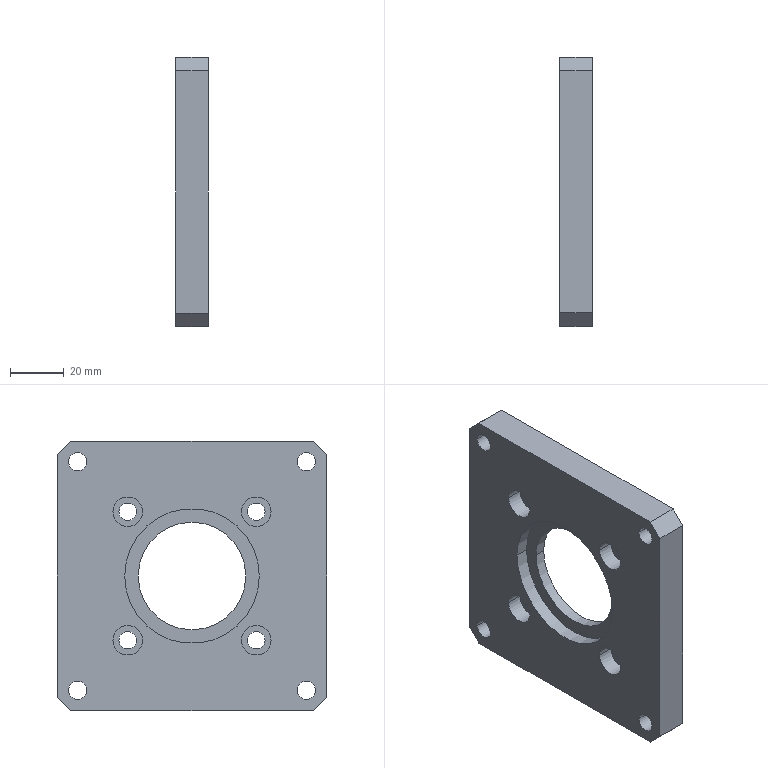Component | SolidWorks | LowerSideBeltXG-XG1-1_MotorMountingPlate-XG1-1 | 1 solid | 46 faces | box 12 x 100 x 100 mm | volume 92608 mm3 | cylinder 30 | plane 16 | commonest cylinder face diameters 6.8 x8 11 x8 6.5 x8 50 x2 55 x2 40 x2
build123d program:
from build123d import *

# Parameters (mm, degrees)
SKETCH1_W                                       = 100
SKETCH1_H                                       = 100
BOSS_EXTRUDE1_DEPTH                             = 12
SKETCH2_R                                       = 27.5
CUT_EXTRUDE1_DEPTH                              = 3
SKETCH3_R                                       = 20
CUT_EXTRUDE2_DEPTH                              = 72.281
SKETCH4_R                                       = 25
CUT_EXTRUDE3_DEPTH                              = 5
M6_HEX_SOCKET_HEAD_CAP_SCREW_CBORE1_D           = 6.5
M6_HEX_SOCKET_HEAD_CAP_SCREW_CBORE1_CBORE_D     = 11
M6_HEX_SOCKET_HEAD_CAP_SCREW_CBORE1_CBORE_DEPTH = 6
M8_TAPPED_HOLE1_D                               = 6.8
CHAMFER1_SIZE                                   = 5


with BuildPart() as part:
    # Sketch1 → Boss-Extrude1 (new body)
    with BuildSketch(Plane.XY):
        Rectangle(SKETCH1_W, SKETCH1_H)
    extrude(amount=BOSS_EXTRUDE1_DEPTH)

    # Sketch2 → Cut-Extrude1 (cut)
    with BuildSketch(Plane.XY.offset(12)):
        Circle(SKETCH2_R)
    extrude(amount=-CUT_EXTRUDE1_DEPTH, mode=Mode.SUBTRACT)

    # Sketch3 → Cut-Extrude2 (cut, through all)
    with BuildSketch(Plane.XY.offset(9)):
        Circle(SKETCH3_R)
    extrude(amount=-CUT_EXTRUDE2_DEPTH, mode=Mode.SUBTRACT)

    # Sketch4 → Cut-Extrude3 (cut)
    with BuildSketch(Plane(origin=(0, 0, 0), x_dir=(-1, 0, 0), z_dir=(0, 0, -1))):
        Circle(SKETCH4_R)
    extrude(amount=-CUT_EXTRUDE3_DEPTH, mode=Mode.SUBTRACT)

    # M6 Hex Socket Head Cap Screw CBORE1 (through all)
    with Locations(Plane(origin=(0, 0, 0), x_dir=(-1, 0, 0), z_dir=(0, 0, -1))):
        with Locations((-23.865, 23.865), (23.865, 23.865), (23.865, -23.865), (-23.865, -23.865)):
            CounterBoreHole(M6_HEX_SOCKET_HEAD_CAP_SCREW_CBORE1_D / 2, M6_HEX_SOCKET_HEAD_CAP_SCREW_CBORE1_CBORE_D / 2, M6_HEX_SOCKET_HEAD_CAP_SCREW_CBORE1_CBORE_DEPTH)

    # M8 Tapped Hole1 (through all)
    with Locations(Plane(origin=(0, 0, 0), x_dir=(-1, 0, 0), z_dir=(0, 0, -1))):
        with Locations((-42.426, 42.426), (-42.426, -42.426), (42.426, -42.426), (42.426, 42.426)):
            Hole(M8_TAPPED_HOLE1_D / 2)

    # Chamfer1
    chamfer1_edges = [part.edges().sort_by_distance(p)[0] for p in [
        (50, -50, 6),
        (-50, -50, 6),
        (-50, 50, 6),
        (50, 50, 6),
    ]]
    chamfer(chamfer1_edges, length=CHAMFER1_SIZE)


solid = part.part

# Placed as in the assembly
solid = solid.moved(Location((-393.22, 625, 114), (0, 90, 0)))